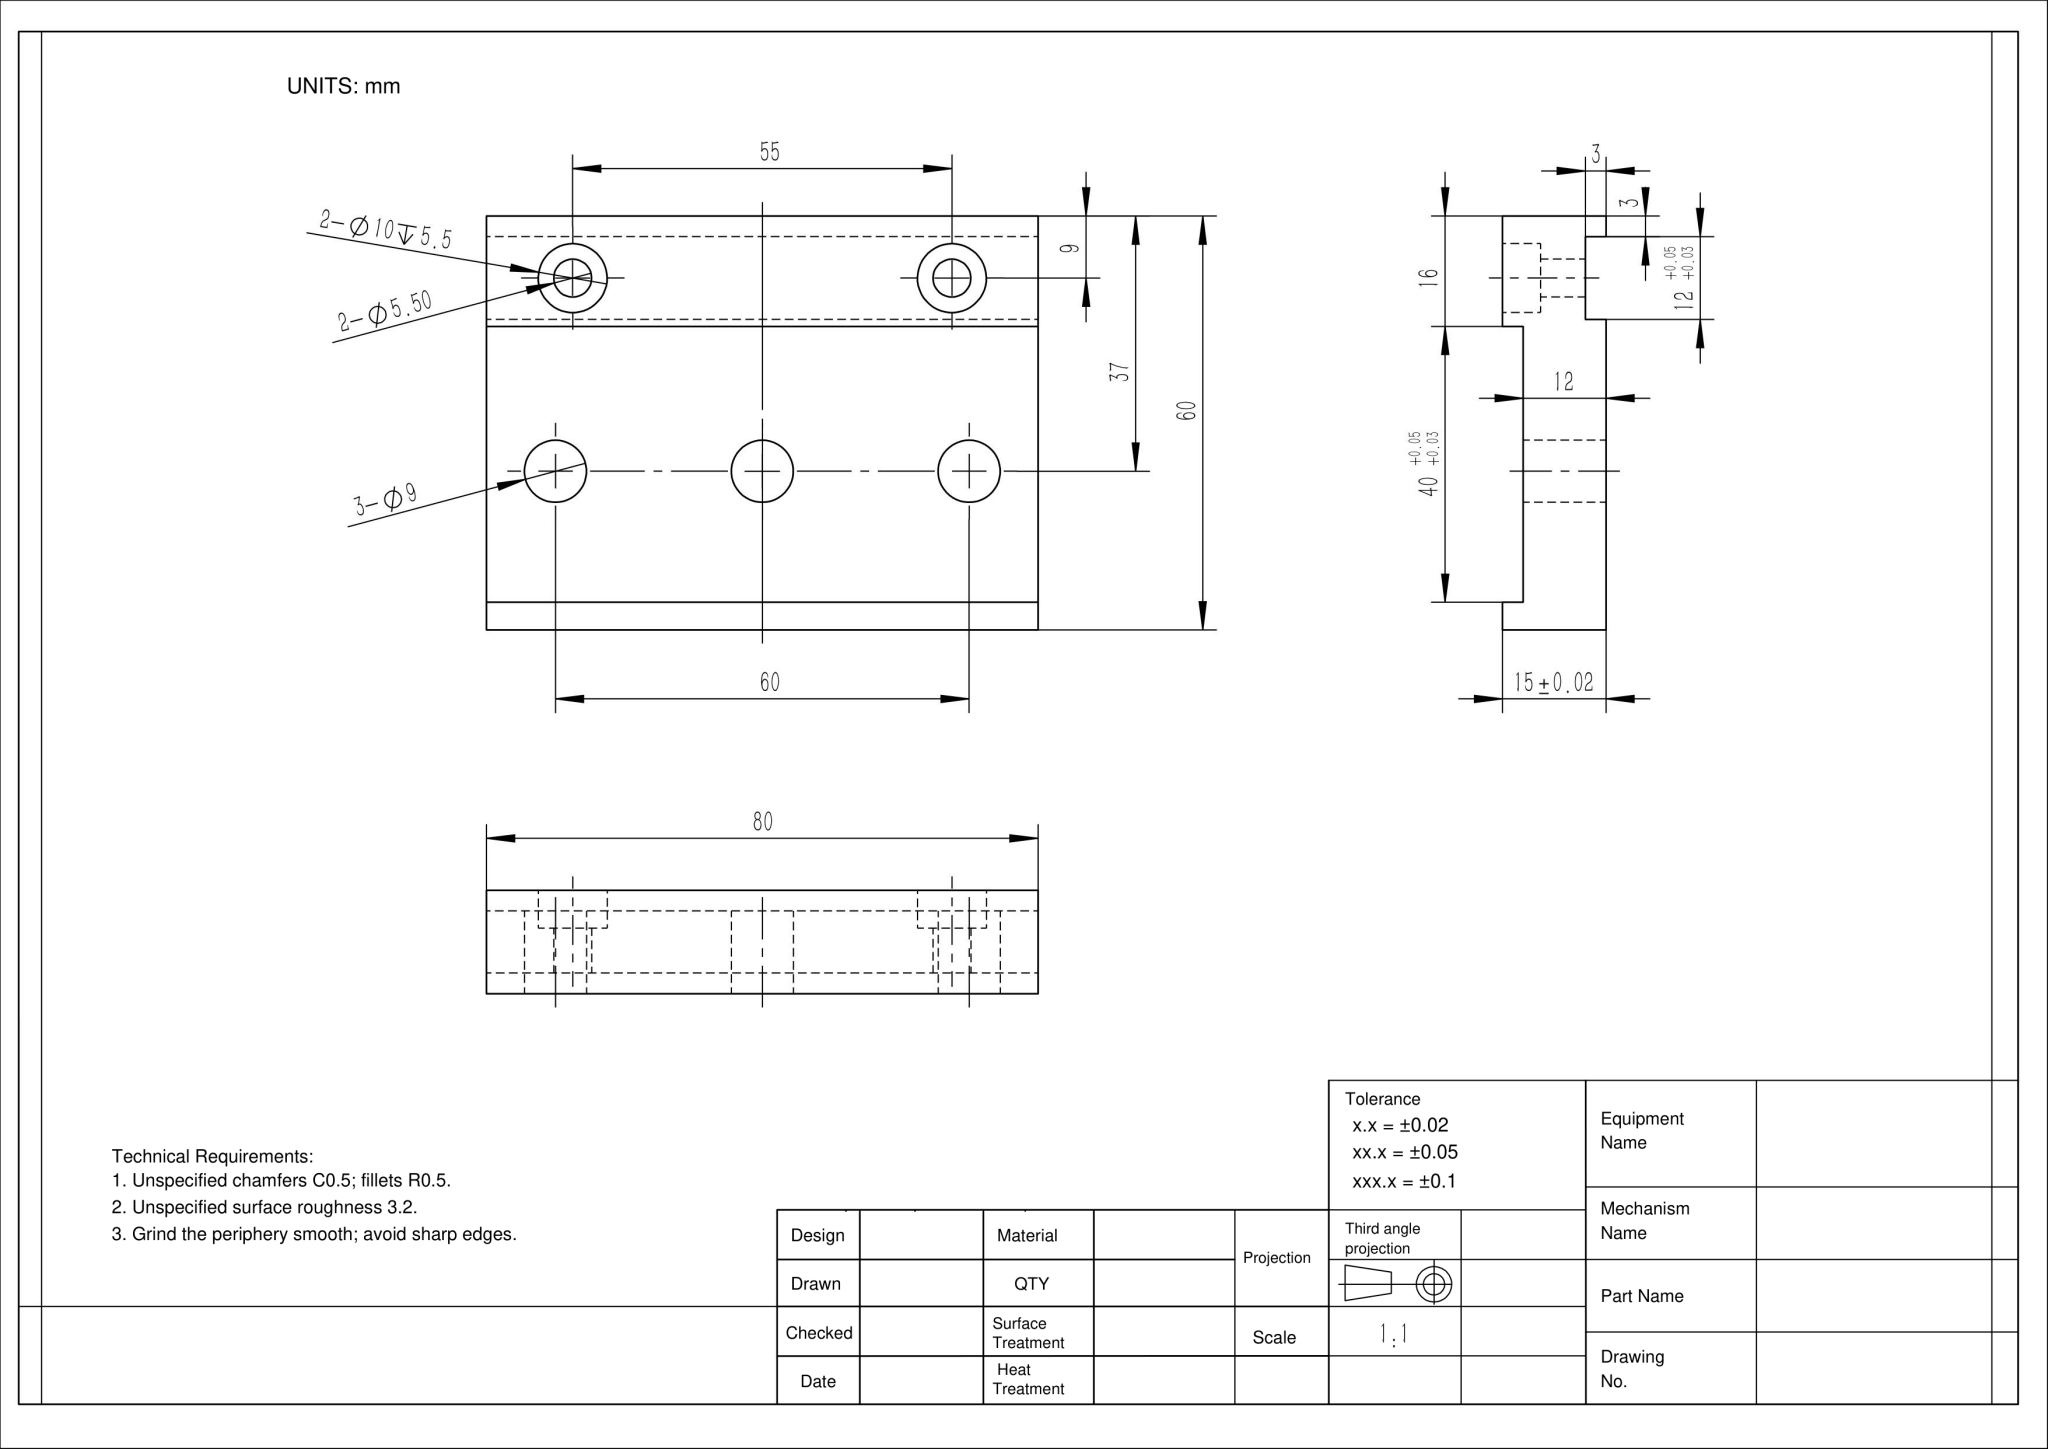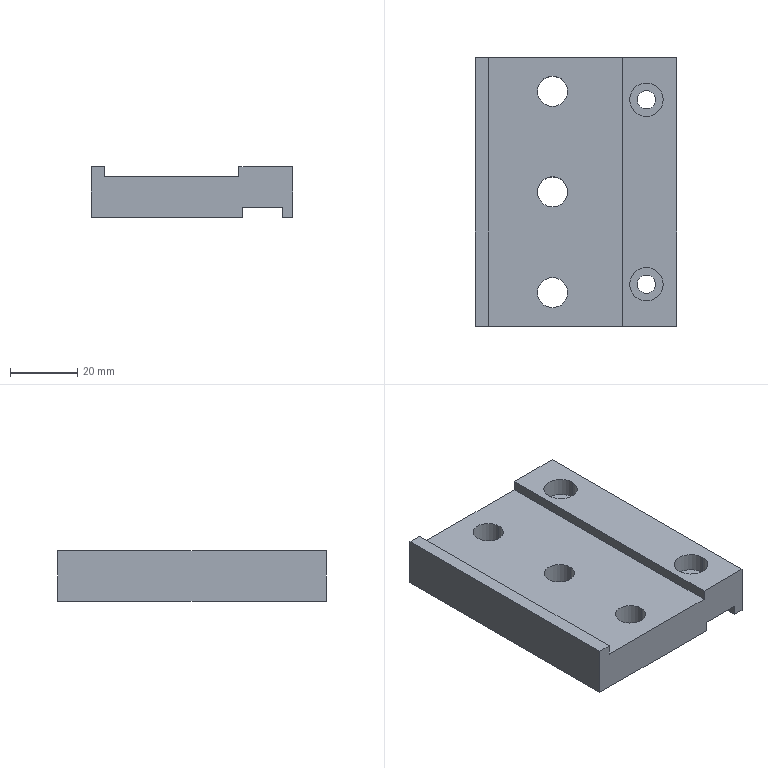Part | NX | mm | 1 solid | 30 faces | box 60 x 80 x 15 mm | volume 56057 mm3 | plane 16 | cylinder 14 | commonest cylinder face diameters 9 x6 10 x4 5.5 x4
STEP:
#1=CARTESIAN_POINT('',(46.,12.5,9.5));
#2=VERTEX_POINT('',#1);
#3=CARTESIAN_POINT('',(56.,12.5,9.5));
#4=VERTEX_POINT('',#3);
#5=CARTESIAN_POINT('',(51.,12.5,9.5));
#6=DIRECTION('',(0.,0.,1.));
#7=DIRECTION('',(1.,0.,0.));
#8=AXIS2_PLACEMENT_3D('',#5,#6,#7);
#9=CIRCLE('',#8,5.);
#10=EDGE_CURVE('',#2,#4,#9,.T.);
#11=ORIENTED_EDGE('',*,*,#10,.F.);
#12=CARTESIAN_POINT('',(46.,12.5,15.));
#13=VERTEX_POINT('',#12);
#14=CARTESIAN_POINT('',(46.,12.5,15.));
#15=DIRECTION('',(0.,0.,1.));
#16=VECTOR('',#15,1000.);
#17=LINE('',#14,#16);
#18=EDGE_CURVE('',#2,#13,#17,.T.);
#19=ORIENTED_EDGE('',*,*,#18,.T.);
#20=CARTESIAN_POINT('',(56.,12.5,15.));
#21=VERTEX_POINT('',#20);
#22=CARTESIAN_POINT('',(51.,12.5,15.));
#23=DIRECTION('',(0.,0.,1.));
#24=DIRECTION('',(1.,0.,0.));
#25=AXIS2_PLACEMENT_3D('',#22,#23,#24);
#26=CIRCLE('',#25,5.);
#27=EDGE_CURVE('',#13,#21,#26,.T.);
#28=ORIENTED_EDGE('',*,*,#27,.T.);
#29=CARTESIAN_POINT('',(56.,12.5,15.));
#30=DIRECTION('',(0.,0.,1.));
#31=VECTOR('',#30,1000.);
#32=LINE('',#29,#31);
#33=EDGE_CURVE('',#4,#21,#32,.T.);
#34=ORIENTED_EDGE('',*,*,#33,.F.);
#35=EDGE_LOOP('',(#11,#19,#28,#34));
#36=FACE_OUTER_BOUND('',#35,.T.);
#37=CARTESIAN_POINT('',(51.,12.5,15.));
#38=DIRECTION('',(0.,0.,1.));
#39=DIRECTION('',(1.,0.,0.));
#40=AXIS2_PLACEMENT_3D('',#37,#38,#39);
#41=CYLINDRICAL_SURFACE('',#40,5.);
#42=ADVANCED_FACE('',(#36),#41,.F.);
#43=CARTESIAN_POINT('',(53.75,12.5,3.));
#44=VERTEX_POINT('',#43);
#45=CARTESIAN_POINT('',(48.25,12.5,3.));
#46=VERTEX_POINT('',#45);
#47=CARTESIAN_POINT('',(51.,12.5,3.));
#48=DIRECTION('',(0.,0.,-1.));
#49=DIRECTION('',(-1.,0.,0.));
#50=AXIS2_PLACEMENT_3D('',#47,#48,#49);
#51=CIRCLE('',#50,2.75);
#52=EDGE_CURVE('',#44,#46,#51,.T.);
#53=ORIENTED_EDGE('',*,*,#52,.T.);
#54=CARTESIAN_POINT('',(48.25,12.5,9.5));
#55=VERTEX_POINT('',#54);
#56=CARTESIAN_POINT('',(48.25,12.5,15.));
#57=DIRECTION('',(0.,0.,1.));
#58=VECTOR('',#57,1000.);
#59=LINE('',#56,#58);
#60=EDGE_CURVE('',#46,#55,#59,.T.);
#61=ORIENTED_EDGE('',*,*,#60,.T.);
#62=CARTESIAN_POINT('',(53.75,12.5,9.5));
#63=VERTEX_POINT('',#62);
#64=CARTESIAN_POINT('',(51.,12.5,9.5));
#65=DIRECTION('',(0.,0.,1.));
#66=DIRECTION('',(1.,0.,0.));
#67=AXIS2_PLACEMENT_3D('',#64,#65,#66);
#68=CIRCLE('',#67,2.75);
#69=EDGE_CURVE('',#55,#63,#68,.T.);
#70=ORIENTED_EDGE('',*,*,#69,.T.);
#71=CARTESIAN_POINT('',(53.75,12.5,15.));
#72=DIRECTION('',(0.,0.,1.));
#73=VECTOR('',#72,1000.);
#74=LINE('',#71,#73);
#75=EDGE_CURVE('',#44,#63,#74,.T.);
#76=ORIENTED_EDGE('',*,*,#75,.F.);
#77=EDGE_LOOP('',(#53,#61,#70,#76));
#78=FACE_OUTER_BOUND('',#77,.T.);
#79=CARTESIAN_POINT('',(51.,12.5,15.));
#80=DIRECTION('',(0.,0.,1.));
#81=DIRECTION('',(1.,0.,0.));
#82=AXIS2_PLACEMENT_3D('',#79,#80,#81);
#83=CYLINDRICAL_SURFACE('',#82,2.75);
#84=ADVANCED_FACE('',(#78),#83,.F.);
#85=CARTESIAN_POINT('',(46.,67.5,9.5));
#86=VERTEX_POINT('',#85);
#87=CARTESIAN_POINT('',(56.,67.5,9.5));
#88=VERTEX_POINT('',#87);
#89=CARTESIAN_POINT('',(51.,67.5,9.5));
#90=DIRECTION('',(0.,0.,1.));
#91=DIRECTION('',(1.,0.,0.));
#92=AXIS2_PLACEMENT_3D('',#89,#90,#91);
#93=CIRCLE('',#92,5.);
#94=EDGE_CURVE('',#86,#88,#93,.T.);
#95=ORIENTED_EDGE('',*,*,#94,.F.);
#96=CARTESIAN_POINT('',(46.,67.5,15.));
#97=VERTEX_POINT('',#96);
#98=CARTESIAN_POINT('',(46.,67.5,15.));
#99=DIRECTION('',(0.,0.,1.));
#100=VECTOR('',#99,1000.);
#101=LINE('',#98,#100);
#102=EDGE_CURVE('',#86,#97,#101,.T.);
#103=ORIENTED_EDGE('',*,*,#102,.T.);
#104=CARTESIAN_POINT('',(56.,67.5,15.));
#105=VERTEX_POINT('',#104);
#106=CARTESIAN_POINT('',(51.,67.5,15.));
#107=DIRECTION('',(0.,0.,1.));
#108=DIRECTION('',(1.,0.,0.));
#109=AXIS2_PLACEMENT_3D('',#106,#107,#108);
#110=CIRCLE('',#109,5.);
#111=EDGE_CURVE('',#97,#105,#110,.T.);
#112=ORIENTED_EDGE('',*,*,#111,.T.);
#113=CARTESIAN_POINT('',(56.,67.5,15.));
#114=DIRECTION('',(0.,0.,1.));
#115=VECTOR('',#114,1000.);
#116=LINE('',#113,#115);
#117=EDGE_CURVE('',#88,#105,#116,.T.);
#118=ORIENTED_EDGE('',*,*,#117,.F.);
#119=EDGE_LOOP('',(#95,#103,#112,#118));
#120=FACE_OUTER_BOUND('',#119,.T.);
#121=CARTESIAN_POINT('',(51.,67.5,15.));
#122=DIRECTION('',(0.,0.,1.));
#123=DIRECTION('',(1.,0.,0.));
#124=AXIS2_PLACEMENT_3D('',#121,#122,#123);
#125=CYLINDRICAL_SURFACE('',#124,5.);
#126=ADVANCED_FACE('',(#120),#125,.F.);
#127=CARTESIAN_POINT('',(53.75,67.5,3.));
#128=VERTEX_POINT('',#127);
#129=CARTESIAN_POINT('',(48.25,67.5,3.));
#130=VERTEX_POINT('',#129);
#131=CARTESIAN_POINT('',(51.,67.5,3.));
#132=DIRECTION('',(0.,0.,-1.));
#133=DIRECTION('',(-1.,0.,0.));
#134=AXIS2_PLACEMENT_3D('',#131,#132,#133);
#135=CIRCLE('',#134,2.75);
#136=EDGE_CURVE('',#128,#130,#135,.T.);
#137=ORIENTED_EDGE('',*,*,#136,.T.);
#138=CARTESIAN_POINT('',(48.25,67.5,9.5));
#139=VERTEX_POINT('',#138);
#140=CARTESIAN_POINT('',(48.25,67.5,15.));
#141=DIRECTION('',(0.,0.,1.));
#142=VECTOR('',#141,1000.);
#143=LINE('',#140,#142);
#144=EDGE_CURVE('',#130,#139,#143,.T.);
#145=ORIENTED_EDGE('',*,*,#144,.T.);
#146=CARTESIAN_POINT('',(53.75,67.5,9.5));
#147=VERTEX_POINT('',#146);
#148=CARTESIAN_POINT('',(51.,67.5,9.5));
#149=DIRECTION('',(0.,0.,1.));
#150=DIRECTION('',(1.,0.,0.));
#151=AXIS2_PLACEMENT_3D('',#148,#149,#150);
#152=CIRCLE('',#151,2.75);
#153=EDGE_CURVE('',#139,#147,#152,.T.);
#154=ORIENTED_EDGE('',*,*,#153,.T.);
#155=CARTESIAN_POINT('',(53.75,67.5,15.));
#156=DIRECTION('',(0.,0.,1.));
#157=VECTOR('',#156,1000.);
#158=LINE('',#155,#157);
#159=EDGE_CURVE('',#128,#147,#158,.T.);
#160=ORIENTED_EDGE('',*,*,#159,.F.);
#161=EDGE_LOOP('',(#137,#145,#154,#160));
#162=FACE_OUTER_BOUND('',#161,.T.);
#163=CARTESIAN_POINT('',(51.,67.5,15.));
#164=DIRECTION('',(0.,0.,1.));
#165=DIRECTION('',(1.,0.,0.));
#166=AXIS2_PLACEMENT_3D('',#163,#164,#165);
#167=CYLINDRICAL_SURFACE('',#166,2.75);
#168=ADVANCED_FACE('',(#162),#167,.F.);
#169=CARTESIAN_POINT('',(18.5,10.,12.));
#170=VERTEX_POINT('',#169);
#171=CARTESIAN_POINT('',(27.5,10.,12.));
#172=VERTEX_POINT('',#171);
#173=CARTESIAN_POINT('',(23.,10.,12.));
#174=DIRECTION('',(0.,0.,1.));
#175=DIRECTION('',(1.,0.,0.));
#176=AXIS2_PLACEMENT_3D('',#173,#174,#175);
#177=CIRCLE('',#176,4.5);
#178=EDGE_CURVE('',#170,#172,#177,.T.);
#179=ORIENTED_EDGE('',*,*,#178,.T.);
#180=CARTESIAN_POINT('',(27.5,10.,-0.));
#181=VERTEX_POINT('',#180);
#182=CARTESIAN_POINT('',(27.5,10.,0.));
#183=DIRECTION('',(0.,0.,-1.));
#184=VECTOR('',#183,1000.);
#185=LINE('',#182,#184);
#186=EDGE_CURVE('',#172,#181,#185,.T.);
#187=ORIENTED_EDGE('',*,*,#186,.T.);
#188=CARTESIAN_POINT('',(18.5,10.,-0.));
#189=VERTEX_POINT('',#188);
#190=CARTESIAN_POINT('',(23.,10.,-0.));
#191=DIRECTION('',(0.,0.,-1.));
#192=DIRECTION('',(-1.,0.,0.));
#193=AXIS2_PLACEMENT_3D('',#190,#191,#192);
#194=CIRCLE('',#193,4.5);
#195=EDGE_CURVE('',#181,#189,#194,.T.);
#196=ORIENTED_EDGE('',*,*,#195,.T.);
#197=CARTESIAN_POINT('',(18.5,10.,0.));
#198=DIRECTION('',(0.,0.,-1.));
#199=VECTOR('',#198,1000.);
#200=LINE('',#197,#199);
#201=EDGE_CURVE('',#170,#189,#200,.T.);
#202=ORIENTED_EDGE('',*,*,#201,.F.);
#203=EDGE_LOOP('',(#179,#187,#196,#202));
#204=FACE_OUTER_BOUND('',#203,.T.);
#205=CARTESIAN_POINT('',(23.,10.,0.));
#206=DIRECTION('',(0.,0.,-1.));
#207=DIRECTION('',(-1.,0.,0.));
#208=AXIS2_PLACEMENT_3D('',#205,#206,#207);
#209=CYLINDRICAL_SURFACE('',#208,4.5);
#210=ADVANCED_FACE('',(#204),#209,.F.);
#211=CARTESIAN_POINT('',(18.5,40.,12.));
#212=VERTEX_POINT('',#211);
#213=CARTESIAN_POINT('',(27.5,40.,12.));
#214=VERTEX_POINT('',#213);
#215=CARTESIAN_POINT('',(23.,40.,12.));
#216=DIRECTION('',(0.,0.,1.));
#217=DIRECTION('',(1.,0.,0.));
#218=AXIS2_PLACEMENT_3D('',#215,#216,#217);
#219=CIRCLE('',#218,4.5);
#220=EDGE_CURVE('',#212,#214,#219,.T.);
#221=ORIENTED_EDGE('',*,*,#220,.T.);
#222=CARTESIAN_POINT('',(27.5,40.,-0.));
#223=VERTEX_POINT('',#222);
#224=CARTESIAN_POINT('',(27.5,40.,0.));
#225=DIRECTION('',(0.,0.,-1.));
#226=VECTOR('',#225,1000.);
#227=LINE('',#224,#226);
#228=EDGE_CURVE('',#214,#223,#227,.T.);
#229=ORIENTED_EDGE('',*,*,#228,.T.);
#230=CARTESIAN_POINT('',(18.5,40.,-0.));
#231=VERTEX_POINT('',#230);
#232=CARTESIAN_POINT('',(23.,40.,-0.));
#233=DIRECTION('',(0.,0.,-1.));
#234=DIRECTION('',(-1.,0.,0.));
#235=AXIS2_PLACEMENT_3D('',#232,#233,#234);
#236=CIRCLE('',#235,4.5);
#237=EDGE_CURVE('',#223,#231,#236,.T.);
#238=ORIENTED_EDGE('',*,*,#237,.T.);
#239=CARTESIAN_POINT('',(18.5,40.,0.));
#240=DIRECTION('',(0.,0.,-1.));
#241=VECTOR('',#240,1000.);
#242=LINE('',#239,#241);
#243=EDGE_CURVE('',#212,#231,#242,.T.);
#244=ORIENTED_EDGE('',*,*,#243,.F.);
#245=EDGE_LOOP('',(#221,#229,#238,#244));
#246=FACE_OUTER_BOUND('',#245,.T.);
#247=CARTESIAN_POINT('',(23.,40.,0.));
#248=DIRECTION('',(0.,0.,-1.));
#249=DIRECTION('',(-1.,0.,0.));
#250=AXIS2_PLACEMENT_3D('',#247,#248,#249);
#251=CYLINDRICAL_SURFACE('',#250,4.5);
#252=ADVANCED_FACE('',(#246),#251,.F.);
#253=CARTESIAN_POINT('',(18.5,70.,12.));
#254=VERTEX_POINT('',#253);
#255=CARTESIAN_POINT('',(27.5,70.,12.));
#256=VERTEX_POINT('',#255);
#257=CARTESIAN_POINT('',(23.,70.,12.));
#258=DIRECTION('',(0.,0.,1.));
#259=DIRECTION('',(1.,0.,0.));
#260=AXIS2_PLACEMENT_3D('',#257,#258,#259);
#261=CIRCLE('',#260,4.5);
#262=EDGE_CURVE('',#254,#256,#261,.T.);
#263=ORIENTED_EDGE('',*,*,#262,.T.);
#264=CARTESIAN_POINT('',(27.5,70.,-0.));
#265=VERTEX_POINT('',#264);
#266=CARTESIAN_POINT('',(27.5,70.,0.));
#267=DIRECTION('',(0.,0.,-1.));
#268=VECTOR('',#267,1000.);
#269=LINE('',#266,#268);
#270=EDGE_CURVE('',#256,#265,#269,.T.);
#271=ORIENTED_EDGE('',*,*,#270,.T.);
#272=CARTESIAN_POINT('',(18.5,70.,-0.));
#273=VERTEX_POINT('',#272);
#274=CARTESIAN_POINT('',(23.,70.,-0.));
#275=DIRECTION('',(0.,0.,-1.));
#276=DIRECTION('',(-1.,0.,0.));
#277=AXIS2_PLACEMENT_3D('',#274,#275,#276);
#278=CIRCLE('',#277,4.5);
#279=EDGE_CURVE('',#265,#273,#278,.T.);
#280=ORIENTED_EDGE('',*,*,#279,.T.);
#281=CARTESIAN_POINT('',(18.5,70.,0.));
#282=DIRECTION('',(0.,0.,-1.));
#283=VECTOR('',#282,1000.);
#284=LINE('',#281,#283);
#285=EDGE_CURVE('',#254,#273,#284,.T.);
#286=ORIENTED_EDGE('',*,*,#285,.F.);
#287=EDGE_LOOP('',(#263,#271,#280,#286));
#288=FACE_OUTER_BOUND('',#287,.T.);
#289=CARTESIAN_POINT('',(23.,70.,0.));
#290=DIRECTION('',(0.,0.,-1.));
#291=DIRECTION('',(-1.,0.,0.));
#292=AXIS2_PLACEMENT_3D('',#289,#290,#291);
#293=CYLINDRICAL_SURFACE('',#292,4.5);
#294=ADVANCED_FACE('',(#288),#293,.F.);
#295=CARTESIAN_POINT('',(57.,80.,0.));
#296=VERTEX_POINT('',#295);
#297=CARTESIAN_POINT('',(57.,0.,0.));
#298=VERTEX_POINT('',#297);
#299=CARTESIAN_POINT('',(57.,80.,0.));
#300=DIRECTION('',(-0.,-1.,0.));
#301=VECTOR('',#300,1000.);
#302=LINE('',#299,#301);
#303=EDGE_CURVE('',#296,#298,#302,.T.);
#304=ORIENTED_EDGE('',*,*,#303,.F.);
#305=CARTESIAN_POINT('',(60.,80.,0.));
#306=VERTEX_POINT('',#305);
#307=CARTESIAN_POINT('',(-0.,80.,0.));
#308=DIRECTION('',(-1.,0.,0.));
#309=VECTOR('',#308,1000.);
#310=LINE('',#307,#309);
#311=EDGE_CURVE('',#306,#296,#310,.T.);
#312=ORIENTED_EDGE('',*,*,#311,.F.);
#313=CARTESIAN_POINT('',(60.,0.,0.));
#314=VERTEX_POINT('',#313);
#315=CARTESIAN_POINT('',(60.,0.,0.));
#316=DIRECTION('',(-0.,1.,0.));
#317=VECTOR('',#316,1000.);
#318=LINE('',#315,#317);
#319=EDGE_CURVE('',#314,#306,#318,.T.);
#320=ORIENTED_EDGE('',*,*,#319,.F.);
#321=CARTESIAN_POINT('',(0.,0.,0.));
#322=DIRECTION('',(1.,0.,0.));
#323=VECTOR('',#322,1000.);
#324=LINE('',#321,#323);
#325=EDGE_CURVE('',#298,#314,#324,.T.);
#326=ORIENTED_EDGE('',*,*,#325,.F.);
#327=EDGE_LOOP('',(#304,#312,#320,#326));
#328=FACE_OUTER_BOUND('',#327,.T.);
#329=CARTESIAN_POINT('',(0.,0.,0.));
#330=DIRECTION('',(0.,0.,-1.));
#331=DIRECTION('',(-1.,0.,0.));
#332=AXIS2_PLACEMENT_3D('',#329,#330,#331);
#333=PLANE('',#332);
#334=ADVANCED_FACE('',(#328),#333,.T.);
#335=CARTESIAN_POINT('',(0.,0.,15.));
#336=VERTEX_POINT('',#335);
#337=CARTESIAN_POINT('',(4.,0.,15.));
#338=VERTEX_POINT('',#337);
#339=CARTESIAN_POINT('',(0.,0.,15.));
#340=DIRECTION('',(1.,0.,0.));
#341=VECTOR('',#340,1000.);
#342=LINE('',#339,#341);
#343=EDGE_CURVE('',#336,#338,#342,.T.);
#344=ORIENTED_EDGE('',*,*,#343,.T.);
#345=CARTESIAN_POINT('',(4.,80.,15.));
#346=VERTEX_POINT('',#345);
#347=CARTESIAN_POINT('',(4.,80.,15.));
#348=DIRECTION('',(0.,-1.,0.));
#349=VECTOR('',#348,1000.);
#350=LINE('',#347,#349);
#351=EDGE_CURVE('',#346,#338,#350,.T.);
#352=ORIENTED_EDGE('',*,*,#351,.F.);
#353=CARTESIAN_POINT('',(-0.,80.,15.));
#354=VERTEX_POINT('',#353);
#355=CARTESIAN_POINT('',(-0.,80.,15.));
#356=DIRECTION('',(-1.,0.,0.));
#357=VECTOR('',#356,1000.);
#358=LINE('',#355,#357);
#359=EDGE_CURVE('',#346,#354,#358,.T.);
#360=ORIENTED_EDGE('',*,*,#359,.T.);
#361=CARTESIAN_POINT('',(0.,0.,15.));
#362=DIRECTION('',(0.,-1.,0.));
#363=VECTOR('',#362,1000.);
#364=LINE('',#361,#363);
#365=EDGE_CURVE('',#354,#336,#364,.T.);
#366=ORIENTED_EDGE('',*,*,#365,.T.);
#367=EDGE_LOOP('',(#344,#352,#360,#366));
#368=FACE_OUTER_BOUND('',#367,.T.);
#369=CARTESIAN_POINT('',(0.,0.,15.));
#370=DIRECTION('',(0.,0.,-1.));
#371=DIRECTION('',(-1.,0.,0.));
#372=AXIS2_PLACEMENT_3D('',#369,#370,#371);
#373=PLANE('',#372);
#374=ADVANCED_FACE('',(#368),#373,.F.);
#375=CARTESIAN_POINT('',(-0.,80.,0.));
#376=VERTEX_POINT('',#375);
#377=CARTESIAN_POINT('',(0.,0.,0.));
#378=VERTEX_POINT('',#377);
#379=CARTESIAN_POINT('',(0.,0.,0.));
#380=DIRECTION('',(0.,-1.,0.));
#381=VECTOR('',#380,1000.);
#382=LINE('',#379,#381);
#383=EDGE_CURVE('',#376,#378,#382,.T.);
#384=ORIENTED_EDGE('',*,*,#383,.T.);
#385=CARTESIAN_POINT('',(0.,0.,15.));
#386=DIRECTION('',(0.,0.,-1.));
#387=VECTOR('',#386,1000.);
#388=LINE('',#385,#387);
#389=EDGE_CURVE('',#336,#378,#388,.T.);
#390=ORIENTED_EDGE('',*,*,#389,.F.);
#391=ORIENTED_EDGE('',*,*,#365,.F.);
#392=CARTESIAN_POINT('',(-0.,80.,15.));
#393=DIRECTION('',(0.,0.,-1.));
#394=VECTOR('',#393,1000.);
#395=LINE('',#392,#394);
#396=EDGE_CURVE('',#354,#376,#395,.T.);
#397=ORIENTED_EDGE('',*,*,#396,.T.);
#398=EDGE_LOOP('',(#384,#390,#391,#397));
#399=FACE_OUTER_BOUND('',#398,.T.);
#400=CARTESIAN_POINT('',(0.,0.,15.));
#401=DIRECTION('',(1.,0.,0.));
#402=DIRECTION('',(-0.,1.,0.));
#403=AXIS2_PLACEMENT_3D('',#400,#401,#402);
#404=PLANE('',#403);
#405=ADVANCED_FACE('',(#399),#404,.F.);
#406=CARTESIAN_POINT('',(57.,0.,3.));
#407=VERTEX_POINT('',#406);
#408=CARTESIAN_POINT('',(45.,0.,3.));
#409=VERTEX_POINT('',#408);
#410=CARTESIAN_POINT('',(57.,0.,3.));
#411=DIRECTION('',(-1.,0.,0.));
#412=VECTOR('',#411,1000.);
#413=LINE('',#410,#412);
#414=EDGE_CURVE('',#407,#409,#413,.T.);
#415=ORIENTED_EDGE('',*,*,#414,.F.);
#416=CARTESIAN_POINT('',(57.,0.,3.));
#417=DIRECTION('',(0.,0.,-1.));
#418=VECTOR('',#417,1000.);
#419=LINE('',#416,#418);
#420=EDGE_CURVE('',#407,#298,#419,.T.);
#421=ORIENTED_EDGE('',*,*,#420,.T.);
#422=ORIENTED_EDGE('',*,*,#325,.T.);
#423=CARTESIAN_POINT('',(60.,0.,15.));
#424=VERTEX_POINT('',#423);
#425=CARTESIAN_POINT('',(60.,0.,15.));
#426=DIRECTION('',(0.,0.,-1.));
#427=VECTOR('',#426,1000.);
#428=LINE('',#425,#427);
#429=EDGE_CURVE('',#424,#314,#428,.T.);
#430=ORIENTED_EDGE('',*,*,#429,.F.);
#431=CARTESIAN_POINT('',(44.,0.,15.));
#432=VERTEX_POINT('',#431);
#433=CARTESIAN_POINT('',(0.,0.,15.));
#434=DIRECTION('',(1.,0.,0.));
#435=VECTOR('',#434,1000.);
#436=LINE('',#433,#435);
#437=EDGE_CURVE('',#432,#424,#436,.T.);
#438=ORIENTED_EDGE('',*,*,#437,.F.);
#439=CARTESIAN_POINT('',(44.,0.,12.));
#440=VERTEX_POINT('',#439);
#441=CARTESIAN_POINT('',(44.,0.,12.));
#442=DIRECTION('',(0.,0.,1.));
#443=VECTOR('',#442,1000.);
#444=LINE('',#441,#443);
#445=EDGE_CURVE('',#440,#432,#444,.T.);
#446=ORIENTED_EDGE('',*,*,#445,.F.);
#447=CARTESIAN_POINT('',(4.,0.,12.));
#448=VERTEX_POINT('',#447);
#449=CARTESIAN_POINT('',(4.,0.,12.));
#450=DIRECTION('',(1.,0.,0.));
#451=VECTOR('',#450,1000.);
#452=LINE('',#449,#451);
#453=EDGE_CURVE('',#448,#440,#452,.T.);
#454=ORIENTED_EDGE('',*,*,#453,.F.);
#455=CARTESIAN_POINT('',(4.,0.,12.));
#456=DIRECTION('',(0.,0.,1.));
#457=VECTOR('',#456,1000.);
#458=LINE('',#455,#457);
#459=EDGE_CURVE('',#448,#338,#458,.T.);
#460=ORIENTED_EDGE('',*,*,#459,.T.);
#461=ORIENTED_EDGE('',*,*,#343,.F.);
#462=ORIENTED_EDGE('',*,*,#389,.T.);
#463=CARTESIAN_POINT('',(45.,0.,0.));
#464=VERTEX_POINT('',#463);
#465=CARTESIAN_POINT('',(0.,0.,0.));
#466=DIRECTION('',(1.,0.,0.));
#467=VECTOR('',#466,1000.);
#468=LINE('',#465,#467);
#469=EDGE_CURVE('',#378,#464,#468,.T.);
#470=ORIENTED_EDGE('',*,*,#469,.T.);
#471=CARTESIAN_POINT('',(45.,0.,3.));
#472=DIRECTION('',(0.,0.,-1.));
#473=VECTOR('',#472,1000.);
#474=LINE('',#471,#473);
#475=EDGE_CURVE('',#409,#464,#474,.T.);
#476=ORIENTED_EDGE('',*,*,#475,.F.);
#477=EDGE_LOOP('',(#415,#421,#422,#430,#438,#446,#454,#460,#461,#462,#470,#476));
#478=FACE_OUTER_BOUND('',#477,.T.);
#479=CARTESIAN_POINT('',(0.,0.,15.));
#480=DIRECTION('',(0.,1.,0.));
#481=DIRECTION('',(0.,0.,1.));
#482=AXIS2_PLACEMENT_3D('',#479,#480,#481);
#483=PLANE('',#482);
#484=ADVANCED_FACE('',(#478),#483,.F.);
#485=ORIENTED_EDGE('',*,*,#319,.T.);
#486=CARTESIAN_POINT('',(60.,80.,15.));
#487=VERTEX_POINT('',#486);
#488=CARTESIAN_POINT('',(60.,80.,15.));
#489=DIRECTION('',(0.,0.,-1.));
#490=VECTOR('',#489,1000.);
#491=LINE('',#488,#490);
#492=EDGE_CURVE('',#487,#306,#491,.T.);
#493=ORIENTED_EDGE('',*,*,#492,.F.);
#494=CARTESIAN_POINT('',(60.,0.,15.));
#495=DIRECTION('',(-0.,1.,0.));
#496=VECTOR('',#495,1000.);
#497=LINE('',#494,#496);
#498=EDGE_CURVE('',#424,#487,#497,.T.);
#499=ORIENTED_EDGE('',*,*,#498,.F.);
#500=ORIENTED_EDGE('',*,*,#429,.T.);
#501=EDGE_LOOP('',(#485,#493,#499,#500));
#502=FACE_OUTER_BOUND('',#501,.T.);
#503=CARTESIAN_POINT('',(60.,0.,15.));
#504=DIRECTION('',(-1.,-0.,0.));
#505=DIRECTION('',(0.,-1.,0.));
#506=AXIS2_PLACEMENT_3D('',#503,#504,#505);
#507=PLANE('',#506);
#508=ADVANCED_FACE('',(#502),#507,.F.);
#509=ORIENTED_EDGE('',*,*,#311,.T.);
#510=CARTESIAN_POINT('',(57.,80.,3.));
#511=VERTEX_POINT('',#510);
#512=CARTESIAN_POINT('',(57.,80.,3.));
#513=DIRECTION('',(0.,0.,-1.));
#514=VECTOR('',#513,1000.);
#515=LINE('',#512,#514);
#516=EDGE_CURVE('',#511,#296,#515,.T.);
#517=ORIENTED_EDGE('',*,*,#516,.F.);
#518=CARTESIAN_POINT('',(45.,80.,3.));
#519=VERTEX_POINT('',#518);
#520=CARTESIAN_POINT('',(57.,80.,3.));
#521=DIRECTION('',(1.,0.,0.));
#522=VECTOR('',#521,1000.);
#523=LINE('',#520,#522);
#524=EDGE_CURVE('',#519,#511,#523,.T.);
#525=ORIENTED_EDGE('',*,*,#524,.F.);
#526=CARTESIAN_POINT('',(45.,80.,0.));
#527=VERTEX_POINT('',#526);
#528=CARTESIAN_POINT('',(45.,80.,3.));
#529=DIRECTION('',(0.,0.,-1.));
#530=VECTOR('',#529,1000.);
#531=LINE('',#528,#530);
#532=EDGE_CURVE('',#519,#527,#531,.T.);
#533=ORIENTED_EDGE('',*,*,#532,.T.);
#534=CARTESIAN_POINT('',(-0.,80.,0.));
#535=DIRECTION('',(-1.,0.,0.));
#536=VECTOR('',#535,1000.);
#537=LINE('',#534,#536);
#538=EDGE_CURVE('',#527,#376,#537,.T.);
#539=ORIENTED_EDGE('',*,*,#538,.T.);
#540=ORIENTED_EDGE('',*,*,#396,.F.);
#541=ORIENTED_EDGE('',*,*,#359,.F.);
#542=CARTESIAN_POINT('',(4.,80.,12.));
#543=VERTEX_POINT('',#542);
#544=CARTESIAN_POINT('',(4.,80.,12.));
#545=DIRECTION('',(0.,0.,1.));
#546=VECTOR('',#545,1000.);
#547=LINE('',#544,#546);
#548=EDGE_CURVE('',#543,#346,#547,.T.);
#549=ORIENTED_EDGE('',*,*,#548,.F.);
#550=CARTESIAN_POINT('',(44.,80.,12.));
#551=VERTEX_POINT('',#550);
#552=CARTESIAN_POINT('',(4.,80.,12.));
#553=DIRECTION('',(-1.,-0.,0.));
#554=VECTOR('',#553,1000.);
#555=LINE('',#552,#554);
#556=EDGE_CURVE('',#551,#543,#555,.T.);
#557=ORIENTED_EDGE('',*,*,#556,.F.);
#558=CARTESIAN_POINT('',(44.,80.,15.));
#559=VERTEX_POINT('',#558);
#560=CARTESIAN_POINT('',(44.,80.,12.));
#561=DIRECTION('',(0.,0.,1.));
#562=VECTOR('',#561,1000.);
#563=LINE('',#560,#562);
#564=EDGE_CURVE('',#551,#559,#563,.T.);
#565=ORIENTED_EDGE('',*,*,#564,.T.);
#566=CARTESIAN_POINT('',(-0.,80.,15.));
#567=DIRECTION('',(-1.,0.,0.));
#568=VECTOR('',#567,1000.);
#569=LINE('',#566,#568);
#570=EDGE_CURVE('',#487,#559,#569,.T.);
#571=ORIENTED_EDGE('',*,*,#570,.F.);
#572=ORIENTED_EDGE('',*,*,#492,.T.);
#573=EDGE_LOOP('',(#509,#517,#525,#533,#539,#540,#541,#549,#557,#565,#571,#572));
#574=FACE_OUTER_BOUND('',#573,.T.);
#575=CARTESIAN_POINT('',(-0.,80.,15.));
#576=DIRECTION('',(0.,-1.,0.));
#577=DIRECTION('',(0.,0.,-1.));
#578=AXIS2_PLACEMENT_3D('',#575,#576,#577);
#579=PLANE('',#578);
#580=ADVANCED_FACE('',(#574),#579,.F.);
#581=CARTESIAN_POINT('',(51.,12.5,15.));
#582=DIRECTION('',(0.,0.,1.));
#583=DIRECTION('',(1.,0.,0.));
#584=AXIS2_PLACEMENT_3D('',#581,#582,#583);
#585=CIRCLE('',#584,5.);
#586=EDGE_CURVE('',#21,#13,#585,.T.);
#587=ORIENTED_EDGE('',*,*,#586,.F.);
#588=ORIENTED_EDGE('',*,*,#27,.F.);
#589=EDGE_LOOP('',(#587,#588));
#590=FACE_BOUND('',#589,.T.);
#591=CARTESIAN_POINT('',(51.,67.5,15.));
#592=DIRECTION('',(0.,0.,1.));
#593=DIRECTION('',(1.,0.,0.));
#594=AXIS2_PLACEMENT_3D('',#591,#592,#593);
#595=CIRCLE('',#594,5.);
#596=EDGE_CURVE('',#105,#97,#595,.T.);
#597=ORIENTED_EDGE('',*,*,#596,.F.);
#598=ORIENTED_EDGE('',*,*,#111,.F.);
#599=EDGE_LOOP('',(#597,#598));
#600=FACE_BOUND('',#599,.T.);
#601=ORIENTED_EDGE('',*,*,#570,.T.);
#602=CARTESIAN_POINT('',(44.,80.,15.));
#603=DIRECTION('',(-0.,1.,0.));
#604=VECTOR('',#603,1000.);
#605=LINE('',#602,#604);
#606=EDGE_CURVE('',#432,#559,#605,.T.);
#607=ORIENTED_EDGE('',*,*,#606,.F.);
#608=ORIENTED_EDGE('',*,*,#437,.T.);
#609=ORIENTED_EDGE('',*,*,#498,.T.);
#610=EDGE_LOOP('',(#601,#607,#608,#609));
#611=FACE_OUTER_BOUND('',#610,.T.);
#612=CARTESIAN_POINT('',(0.,0.,15.));
#613=DIRECTION('',(0.,0.,-1.));
#614=DIRECTION('',(-1.,0.,0.));
#615=AXIS2_PLACEMENT_3D('',#612,#613,#614);
#616=PLANE('',#615);
#617=ADVANCED_FACE('',(#590,#600,#611),#616,.F.);
#618=CARTESIAN_POINT('',(23.,40.,-0.));
#619=DIRECTION('',(0.,0.,-1.));
#620=DIRECTION('',(-1.,0.,0.));
#621=AXIS2_PLACEMENT_3D('',#618,#619,#620);
#622=CIRCLE('',#621,4.5);
#623=EDGE_CURVE('',#231,#223,#622,.T.);
#624=ORIENTED_EDGE('',*,*,#623,.F.);
#625=ORIENTED_EDGE('',*,*,#237,.F.);
#626=EDGE_LOOP('',(#624,#625));
#627=FACE_BOUND('',#626,.T.);
#628=CARTESIAN_POINT('',(23.,70.,-0.));
#629=DIRECTION('',(0.,0.,-1.));
#630=DIRECTION('',(-1.,0.,0.));
#631=AXIS2_PLACEMENT_3D('',#628,#629,#630);
#632=CIRCLE('',#631,4.5);
#633=EDGE_CURVE('',#273,#265,#632,.T.);
#634=ORIENTED_EDGE('',*,*,#633,.F.);
#635=ORIENTED_EDGE('',*,*,#279,.F.);
#636=EDGE_LOOP('',(#634,#635));
#637=FACE_BOUND('',#636,.T.);
#638=CARTESIAN_POINT('',(45.,80.,0.));
#639=DIRECTION('',(0.,1.,0.));
#640=VECTOR('',#639,1000.);
#641=LINE('',#638,#640);
#642=EDGE_CURVE('',#464,#527,#641,.T.);
#643=ORIENTED_EDGE('',*,*,#642,.F.);
#644=ORIENTED_EDGE('',*,*,#469,.F.);
#645=ORIENTED_EDGE('',*,*,#383,.F.);
#646=ORIENTED_EDGE('',*,*,#538,.F.);
#647=EDGE_LOOP('',(#643,#644,#645,#646));
#648=FACE_OUTER_BOUND('',#647,.T.);
#649=CARTESIAN_POINT('',(23.,10.,-0.));
#650=DIRECTION('',(0.,0.,-1.));
#651=DIRECTION('',(-1.,0.,0.));
#652=AXIS2_PLACEMENT_3D('',#649,#650,#651);
#653=CIRCLE('',#652,4.5);
#654=EDGE_CURVE('',#189,#181,#653,.T.);
#655=ORIENTED_EDGE('',*,*,#654,.F.);
#656=ORIENTED_EDGE('',*,*,#195,.F.);
#657=EDGE_LOOP('',(#655,#656));
#658=FACE_BOUND('',#657,.T.);
#659=CARTESIAN_POINT('',(0.,0.,0.));
#660=DIRECTION('',(0.,0.,-1.));
#661=DIRECTION('',(-1.,0.,0.));
#662=AXIS2_PLACEMENT_3D('',#659,#660,#661);
#663=PLANE('',#662);
#664=ADVANCED_FACE('',(#627,#637,#648,#658),#663,.T.);
#665=ORIENTED_EDGE('',*,*,#351,.T.);
#666=ORIENTED_EDGE('',*,*,#459,.F.);
#667=CARTESIAN_POINT('',(4.,80.,12.));
#668=DIRECTION('',(0.,-1.,0.));
#669=VECTOR('',#668,1000.);
#670=LINE('',#667,#669);
#671=EDGE_CURVE('',#543,#448,#670,.T.);
#672=ORIENTED_EDGE('',*,*,#671,.F.);
#673=ORIENTED_EDGE('',*,*,#548,.T.);
#674=EDGE_LOOP('',(#665,#666,#672,#673));
#675=FACE_OUTER_BOUND('',#674,.T.);
#676=CARTESIAN_POINT('',(4.,80.,12.));
#677=DIRECTION('',(-1.,-0.,0.));
#678=DIRECTION('',(0.,-1.,0.));
#679=AXIS2_PLACEMENT_3D('',#676,#677,#678);
#680=PLANE('',#679);
#681=ADVANCED_FACE('',(#675),#680,.F.);
#682=ORIENTED_EDGE('',*,*,#606,.T.);
#683=ORIENTED_EDGE('',*,*,#564,.F.);
#684=CARTESIAN_POINT('',(44.,80.,12.));
#685=DIRECTION('',(-0.,1.,0.));
#686=VECTOR('',#685,1000.);
#687=LINE('',#684,#686);
#688=EDGE_CURVE('',#440,#551,#687,.T.);
#689=ORIENTED_EDGE('',*,*,#688,.F.);
#690=ORIENTED_EDGE('',*,*,#445,.T.);
#691=EDGE_LOOP('',(#682,#683,#689,#690));
#692=FACE_OUTER_BOUND('',#691,.T.);
#693=CARTESIAN_POINT('',(44.,80.,12.));
#694=DIRECTION('',(1.,0.,0.));
#695=DIRECTION('',(-0.,1.,0.));
#696=AXIS2_PLACEMENT_3D('',#693,#694,#695);
#697=PLANE('',#696);
#698=ADVANCED_FACE('',(#692),#697,.F.);
#699=ORIENTED_EDGE('',*,*,#220,.F.);
#700=CARTESIAN_POINT('',(23.,40.,12.));
#701=DIRECTION('',(0.,0.,1.));
#702=DIRECTION('',(1.,0.,0.));
#703=AXIS2_PLACEMENT_3D('',#700,#701,#702);
#704=CIRCLE('',#703,4.5);
#705=EDGE_CURVE('',#214,#212,#704,.T.);
#706=ORIENTED_EDGE('',*,*,#705,.F.);
#707=EDGE_LOOP('',(#699,#706));
#708=FACE_BOUND('',#707,.T.);
#709=ORIENTED_EDGE('',*,*,#262,.F.);
#710=CARTESIAN_POINT('',(23.,70.,12.));
#711=DIRECTION('',(0.,0.,1.));
#712=DIRECTION('',(1.,0.,0.));
#713=AXIS2_PLACEMENT_3D('',#710,#711,#712);
#714=CIRCLE('',#713,4.5);
#715=EDGE_CURVE('',#256,#254,#714,.T.);
#716=ORIENTED_EDGE('',*,*,#715,.F.);
#717=EDGE_LOOP('',(#709,#716));
#718=FACE_BOUND('',#717,.T.);
#719=ORIENTED_EDGE('',*,*,#671,.T.);
#720=ORIENTED_EDGE('',*,*,#453,.T.);
#721=ORIENTED_EDGE('',*,*,#688,.T.);
#722=ORIENTED_EDGE('',*,*,#556,.T.);
#723=EDGE_LOOP('',(#719,#720,#721,#722));
#724=FACE_OUTER_BOUND('',#723,.T.);
#725=ORIENTED_EDGE('',*,*,#178,.F.);
#726=CARTESIAN_POINT('',(23.,10.,12.));
#727=DIRECTION('',(0.,0.,1.));
#728=DIRECTION('',(1.,0.,0.));
#729=AXIS2_PLACEMENT_3D('',#726,#727,#728);
#730=CIRCLE('',#729,4.5);
#731=EDGE_CURVE('',#172,#170,#730,.T.);
#732=ORIENTED_EDGE('',*,*,#731,.F.);
#733=EDGE_LOOP('',(#725,#732));
#734=FACE_BOUND('',#733,.T.);
#735=CARTESIAN_POINT('',(0.,0.,12.));
#736=DIRECTION('',(0.,0.,1.));
#737=DIRECTION('',(1.,0.,0.));
#738=AXIS2_PLACEMENT_3D('',#735,#736,#737);
#739=PLANE('',#738);
#740=ADVANCED_FACE('',(#708,#718,#724,#734),#739,.T.);
#741=ORIENTED_EDGE('',*,*,#303,.T.);
#742=ORIENTED_EDGE('',*,*,#420,.F.);
#743=CARTESIAN_POINT('',(57.,80.,3.));
#744=DIRECTION('',(-0.,-1.,0.));
#745=VECTOR('',#744,1000.);
#746=LINE('',#743,#745);
#747=EDGE_CURVE('',#511,#407,#746,.T.);
#748=ORIENTED_EDGE('',*,*,#747,.F.);
#749=ORIENTED_EDGE('',*,*,#516,.T.);
#750=EDGE_LOOP('',(#741,#742,#748,#749));
#751=FACE_OUTER_BOUND('',#750,.T.);
#752=CARTESIAN_POINT('',(57.,80.,3.));
#753=DIRECTION('',(1.,-0.,0.));
#754=DIRECTION('',(0.,1.,0.));
#755=AXIS2_PLACEMENT_3D('',#752,#753,#754);
#756=PLANE('',#755);
#757=ADVANCED_FACE('',(#751),#756,.F.);
#758=ORIENTED_EDGE('',*,*,#642,.T.);
#759=ORIENTED_EDGE('',*,*,#532,.F.);
#760=CARTESIAN_POINT('',(45.,80.,3.));
#761=DIRECTION('',(0.,1.,0.));
#762=VECTOR('',#761,1000.);
#763=LINE('',#760,#762);
#764=EDGE_CURVE('',#409,#519,#763,.T.);
#765=ORIENTED_EDGE('',*,*,#764,.F.);
#766=ORIENTED_EDGE('',*,*,#475,.T.);
#767=EDGE_LOOP('',(#758,#759,#765,#766));
#768=FACE_OUTER_BOUND('',#767,.T.);
#769=CARTESIAN_POINT('',(45.,80.,3.));
#770=DIRECTION('',(-1.,0.,0.));
#771=DIRECTION('',(-0.,-1.,0.));
#772=AXIS2_PLACEMENT_3D('',#769,#770,#771);
#773=PLANE('',#772);
#774=ADVANCED_FACE('',(#768),#773,.F.);
#775=ORIENTED_EDGE('',*,*,#52,.F.);
#776=CARTESIAN_POINT('',(51.,12.5,3.));
#777=DIRECTION('',(0.,0.,-1.));
#778=DIRECTION('',(-1.,0.,0.));
#779=AXIS2_PLACEMENT_3D('',#776,#777,#778);
#780=CIRCLE('',#779,2.75);
#781=EDGE_CURVE('',#46,#44,#780,.T.);
#782=ORIENTED_EDGE('',*,*,#781,.F.);
#783=EDGE_LOOP('',(#775,#782));
#784=FACE_BOUND('',#783,.T.);
#785=ORIENTED_EDGE('',*,*,#136,.F.);
#786=CARTESIAN_POINT('',(51.,67.5,3.));
#787=DIRECTION('',(0.,0.,-1.));
#788=DIRECTION('',(-1.,0.,0.));
#789=AXIS2_PLACEMENT_3D('',#786,#787,#788);
#790=CIRCLE('',#789,2.75);
#791=EDGE_CURVE('',#130,#128,#790,.T.);
#792=ORIENTED_EDGE('',*,*,#791,.F.);
#793=EDGE_LOOP('',(#785,#792));
#794=FACE_BOUND('',#793,.T.);
#795=ORIENTED_EDGE('',*,*,#747,.T.);
#796=ORIENTED_EDGE('',*,*,#414,.T.);
#797=ORIENTED_EDGE('',*,*,#764,.T.);
#798=ORIENTED_EDGE('',*,*,#524,.T.);
#799=EDGE_LOOP('',(#795,#796,#797,#798));
#800=FACE_OUTER_BOUND('',#799,.T.);
#801=CARTESIAN_POINT('',(0.,0.,3.));
#802=DIRECTION('',(0.,0.,-1.));
#803=DIRECTION('',(-1.,0.,0.));
#804=AXIS2_PLACEMENT_3D('',#801,#802,#803);
#805=PLANE('',#804);
#806=ADVANCED_FACE('',(#784,#794,#800),#805,.T.);
#807=ORIENTED_EDGE('',*,*,#270,.F.);
#808=ORIENTED_EDGE('',*,*,#715,.T.);
#809=ORIENTED_EDGE('',*,*,#285,.T.);
#810=ORIENTED_EDGE('',*,*,#633,.T.);
#811=EDGE_LOOP('',(#807,#808,#809,#810));
#812=FACE_OUTER_BOUND('',#811,.T.);
#813=CARTESIAN_POINT('',(23.,70.,0.));
#814=DIRECTION('',(0.,0.,-1.));
#815=DIRECTION('',(-1.,0.,0.));
#816=AXIS2_PLACEMENT_3D('',#813,#814,#815);
#817=CYLINDRICAL_SURFACE('',#816,4.5);
#818=ADVANCED_FACE('',(#812),#817,.F.);
#819=ORIENTED_EDGE('',*,*,#228,.F.);
#820=ORIENTED_EDGE('',*,*,#705,.T.);
#821=ORIENTED_EDGE('',*,*,#243,.T.);
#822=ORIENTED_EDGE('',*,*,#623,.T.);
#823=EDGE_LOOP('',(#819,#820,#821,#822));
#824=FACE_OUTER_BOUND('',#823,.T.);
#825=CARTESIAN_POINT('',(23.,40.,0.));
#826=DIRECTION('',(0.,0.,-1.));
#827=DIRECTION('',(-1.,0.,0.));
#828=AXIS2_PLACEMENT_3D('',#825,#826,#827);
#829=CYLINDRICAL_SURFACE('',#828,4.5);
#830=ADVANCED_FACE('',(#824),#829,.F.);
#831=ORIENTED_EDGE('',*,*,#186,.F.);
#832=ORIENTED_EDGE('',*,*,#731,.T.);
#833=ORIENTED_EDGE('',*,*,#201,.T.);
#834=ORIENTED_EDGE('',*,*,#654,.T.);
#835=EDGE_LOOP('',(#831,#832,#833,#834));
#836=FACE_OUTER_BOUND('',#835,.T.);
#837=CARTESIAN_POINT('',(23.,10.,0.));
#838=DIRECTION('',(0.,0.,-1.));
#839=DIRECTION('',(-1.,0.,0.));
#840=AXIS2_PLACEMENT_3D('',#837,#838,#839);
#841=CYLINDRICAL_SURFACE('',#840,4.5);
#842=ADVANCED_FACE('',(#836),#841,.F.);
#843=ORIENTED_EDGE('',*,*,#144,.F.);
#844=ORIENTED_EDGE('',*,*,#791,.T.);
#845=ORIENTED_EDGE('',*,*,#159,.T.);
#846=CARTESIAN_POINT('',(51.,67.5,9.5));
#847=DIRECTION('',(0.,0.,1.));
#848=DIRECTION('',(1.,0.,0.));
#849=AXIS2_PLACEMENT_3D('',#846,#847,#848);
#850=CIRCLE('',#849,2.75);
#851=EDGE_CURVE('',#147,#139,#850,.T.);
#852=ORIENTED_EDGE('',*,*,#851,.T.);
#853=EDGE_LOOP('',(#843,#844,#845,#852));
#854=FACE_OUTER_BOUND('',#853,.T.);
#855=CARTESIAN_POINT('',(51.,67.5,15.));
#856=DIRECTION('',(0.,0.,1.));
#857=DIRECTION('',(1.,0.,0.));
#858=AXIS2_PLACEMENT_3D('',#855,#856,#857);
#859=CYLINDRICAL_SURFACE('',#858,2.75);
#860=ADVANCED_FACE('',(#854),#859,.F.);
#861=ORIENTED_EDGE('',*,*,#851,.F.);
#862=ORIENTED_EDGE('',*,*,#153,.F.);
#863=EDGE_LOOP('',(#861,#862));
#864=FACE_BOUND('',#863,.T.);
#865=CARTESIAN_POINT('',(51.,67.5,9.5));
#866=DIRECTION('',(0.,0.,1.));
#867=DIRECTION('',(1.,0.,0.));
#868=AXIS2_PLACEMENT_3D('',#865,#866,#867);
#869=CIRCLE('',#868,5.);
#870=EDGE_CURVE('',#88,#86,#869,.T.);
#871=ORIENTED_EDGE('',*,*,#870,.T.);
#872=ORIENTED_EDGE('',*,*,#94,.T.);
#873=EDGE_LOOP('',(#871,#872));
#874=FACE_OUTER_BOUND('',#873,.T.);
#875=CARTESIAN_POINT('',(53.75,67.5,9.5));
#876=DIRECTION('',(0.,0.,-1.));
#877=DIRECTION('',(-1.,0.,0.));
#878=AXIS2_PLACEMENT_3D('',#875,#876,#877);
#879=PLANE('',#878);
#880=ADVANCED_FACE('',(#864,#874),#879,.F.);
#881=ORIENTED_EDGE('',*,*,#102,.F.);
#882=ORIENTED_EDGE('',*,*,#870,.F.);
#883=ORIENTED_EDGE('',*,*,#117,.T.);
#884=ORIENTED_EDGE('',*,*,#596,.T.);
#885=EDGE_LOOP('',(#881,#882,#883,#884));
#886=FACE_OUTER_BOUND('',#885,.T.);
#887=CARTESIAN_POINT('',(51.,67.5,15.));
#888=DIRECTION('',(0.,0.,1.));
#889=DIRECTION('',(1.,0.,0.));
#890=AXIS2_PLACEMENT_3D('',#887,#888,#889);
#891=CYLINDRICAL_SURFACE('',#890,5.);
#892=ADVANCED_FACE('',(#886),#891,.F.);
#893=ORIENTED_EDGE('',*,*,#60,.F.);
#894=ORIENTED_EDGE('',*,*,#781,.T.);
#895=ORIENTED_EDGE('',*,*,#75,.T.);
#896=CARTESIAN_POINT('',(51.,12.5,9.5));
#897=DIRECTION('',(0.,0.,1.));
#898=DIRECTION('',(1.,0.,0.));
#899=AXIS2_PLACEMENT_3D('',#896,#897,#898);
#900=CIRCLE('',#899,2.75);
#901=EDGE_CURVE('',#63,#55,#900,.T.);
#902=ORIENTED_EDGE('',*,*,#901,.T.);
#903=EDGE_LOOP('',(#893,#894,#895,#902));
#904=FACE_OUTER_BOUND('',#903,.T.);
#905=CARTESIAN_POINT('',(51.,12.5,15.));
#906=DIRECTION('',(0.,0.,1.));
#907=DIRECTION('',(1.,0.,0.));
#908=AXIS2_PLACEMENT_3D('',#905,#906,#907);
#909=CYLINDRICAL_SURFACE('',#908,2.75);
#910=ADVANCED_FACE('',(#904),#909,.F.);
#911=ORIENTED_EDGE('',*,*,#901,.F.);
#912=ORIENTED_EDGE('',*,*,#69,.F.);
#913=EDGE_LOOP('',(#911,#912));
#914=FACE_BOUND('',#913,.T.);
#915=CARTESIAN_POINT('',(51.,12.5,9.5));
#916=DIRECTION('',(0.,0.,1.));
#917=DIRECTION('',(1.,0.,0.));
#918=AXIS2_PLACEMENT_3D('',#915,#916,#917);
#919=CIRCLE('',#918,5.);
#920=EDGE_CURVE('',#4,#2,#919,.T.);
#921=ORIENTED_EDGE('',*,*,#920,.T.);
#922=ORIENTED_EDGE('',*,*,#10,.T.);
#923=EDGE_LOOP('',(#921,#922));
#924=FACE_OUTER_BOUND('',#923,.T.);
#925=CARTESIAN_POINT('',(53.75,12.5,9.5));
#926=DIRECTION('',(0.,0.,-1.));
#927=DIRECTION('',(-1.,0.,0.));
#928=AXIS2_PLACEMENT_3D('',#925,#926,#927);
#929=PLANE('',#928);
#930=ADVANCED_FACE('',(#914,#924),#929,.F.);
#931=ORIENTED_EDGE('',*,*,#18,.F.);
#932=ORIENTED_EDGE('',*,*,#920,.F.);
#933=ORIENTED_EDGE('',*,*,#33,.T.);
#934=ORIENTED_EDGE('',*,*,#586,.T.);
#935=EDGE_LOOP('',(#931,#932,#933,#934));
#936=FACE_OUTER_BOUND('',#935,.T.);
#937=CARTESIAN_POINT('',(51.,12.5,15.));
#938=DIRECTION('',(0.,0.,1.));
#939=DIRECTION('',(1.,0.,0.));
#940=AXIS2_PLACEMENT_3D('',#937,#938,#939);
#941=CYLINDRICAL_SURFACE('',#940,5.);
#942=ADVANCED_FACE('',(#936),#941,.F.);
#943=CLOSED_SHELL('',(#42,#84,#126,#168,#210,#252,#294,#334,#374,#405,#484,#508,#580,#617,#664,#681,#698,#740,#757,#774,#806,#818,#830,#842,#860,#880,#892,#910,#930,#942));
#944=MANIFOLD_SOLID_BREP('',#943);
#945=CARTESIAN_POINT('',(0.,0.,0.));
#946=DIRECTION('',(0.,0.,1.));
#947=DIRECTION('',(1.,0.,0.));
#948=AXIS2_PLACEMENT_3D('',#945,#946,#947);
#949=(LENGTH_UNIT()NAMED_UNIT(*)SI_UNIT(.MILLI.,.METRE.));
#950=UNCERTAINTY_MEASURE_WITH_UNIT(LENGTH_MEASURE(0.00001),#949,'','');
#951=(NAMED_UNIT(*)PLANE_ANGLE_UNIT()SI_UNIT($,.RADIAN.));
#952=(NAMED_UNIT(*)SI_UNIT($,.STERADIAN.)SOLID_ANGLE_UNIT());
#953=(GEOMETRIC_REPRESENTATION_CONTEXT(3)GLOBAL_UNCERTAINTY_ASSIGNED_CONTEXT((#950))GLOBAL_UNIT_ASSIGNED_CONTEXT((#949,#951,#952))REPRESENTATION_CONTEXT('',''));
#954=ADVANCED_BREP_SHAPE_REPRESENTATION('',(#944,#948),#953);
#955=COLOUR_RGB('',0.7922,0.8196,0.9333);
#956=FILL_AREA_STYLE_COLOUR('',#955);
#957=FILL_AREA_STYLE('',(#956));
#958=SURFACE_STYLE_FILL_AREA(#957);
#959=SURFACE_SIDE_STYLE('',(#958));
#960=SURFACE_STYLE_USAGE(.BOTH.,#959);
#961=PRESENTATION_STYLE_ASSIGNMENT((#960));
#962=STYLED_ITEM('',(#961),#944);
#963=(LENGTH_UNIT()NAMED_UNIT(*)SI_UNIT(.MILLI.,.METRE.));
#964=UNCERTAINTY_MEASURE_WITH_UNIT(LENGTH_MEASURE(0.00001),#963,'','');
#965=(NAMED_UNIT(*)PLANE_ANGLE_UNIT()SI_UNIT($,.RADIAN.));
#966=(NAMED_UNIT(*)SI_UNIT($,.STERADIAN.)SOLID_ANGLE_UNIT());
#967=(GEOMETRIC_REPRESENTATION_CONTEXT(3)GLOBAL_UNCERTAINTY_ASSIGNED_CONTEXT((#964))GLOBAL_UNIT_ASSIGNED_CONTEXT((#963,#965,#966))REPRESENTATION_CONTEXT('',''));
#968=MECHANICAL_DESIGN_GEOMETRIC_PRESENTATION_REPRESENTATION('',(#962),#967);
#969=PRESENTATION_LAYER_ASSIGNMENT('','',(#962));